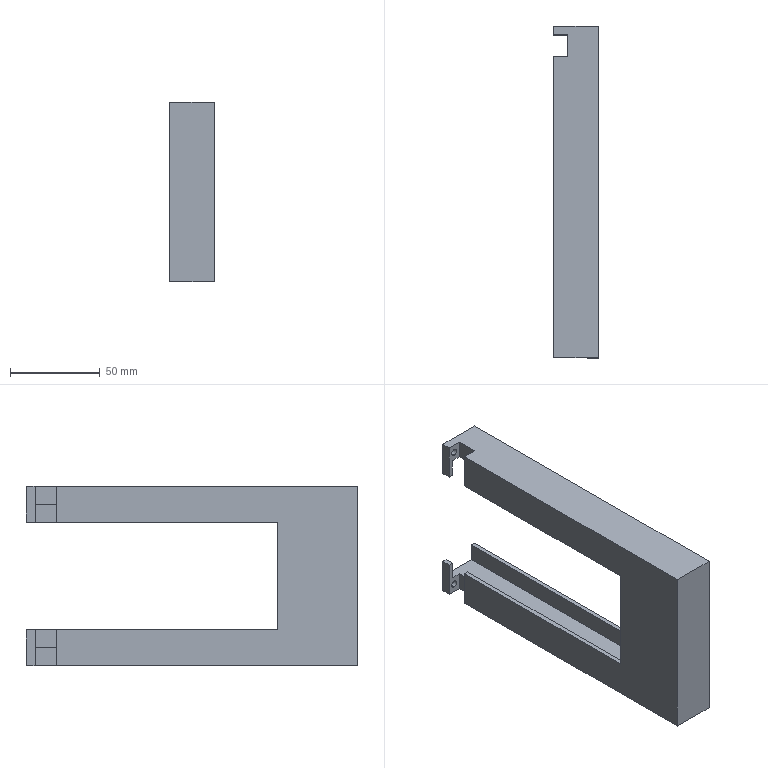Component | SolidWorks | LocatingDie-1_LocatingDieHolder-1 | 1 solid | 34 faces | box 25 x 185 x 100 mm | volume 193854 mm3 | plane 30 | cylinder 4 | commonest cylinder face diameters 4 x4
build123d program:
from build123d import *

# Parameters (mm, degrees)
EXTRUDE1_DEPTH = 25
SKETCH2_W      = 80
SKETCH2_H      = 20
EXTRUDE2_DEPTH = 140
EXTRUDE3_REACH = 140.496
SKETCH3_W      = 8
SKETCH3_H      = 12
EXTRUDE4_REACH = 195.261
SKETCH4_R      = 2


with BuildPart() as part:
    # Sketch1 → Extrude1 (new body)
    with BuildSketch(Plane.XY):
        Polygon((-30, 92.5), (-30, -47.5), (30, -47.5), (30, 92.5), (50, 92.5), (50, -92.5), (-50, -92.5), (-50, 92.5), align=None)
    extrude(amount=EXTRUDE1_DEPTH)

    # Sketch2 → Extrude2 (cut)
    with BuildSketch(Plane(origin=(0, 92.5, 0), x_dir=(1, 0, 0), z_dir=(0, 1, 0))):
        with Locations((0, -12.5)):
            Rectangle(SKETCH2_W, SKETCH2_H)
    extrude(amount=-EXTRUDE2_DEPTH, mode=Mode.SUBTRACT)

    # Extrude3: up to this face of the body (flat: up to its plane)
    extrude3_end = Plane(part.part.faces().sort_by_distance((-50, 0, 12.5))[0])
    # Sketch3 → Extrude3 (cut, up to the picked face)
    with BuildSketch(Plane(origin=(50, 0, 0), x_dir=(0, 0, -1), z_dir=(1, 0, 0)), mode=Mode.PRIVATE) as extrude3_sk1:
        with Locations((-21, 81.5)):
            Rectangle(SKETCH3_W, SKETCH3_H)
    extrude3_tool1 = split(extrude(extrude3_sk1.sketch, amount=-EXTRUDE3_REACH, mode=Mode.PRIVATE), bisect_by=extrude3_end, keep=Keep.BOTH, mode=Mode.PRIVATE)
    add(extrude3_tool1.solids().sort_by(Axis((50, 81.5, 21), (-1, 0, 0)))[0], mode=Mode.SUBTRACT)

    # Sketch4 → Extrude4 (cut, up to next)
    with BuildSketch(Plane(origin=(0, 92.5, 0), x_dir=(1, 0, 0), z_dir=(0, 1, 0)), mode=Mode.PRIVATE) as extrude4_sk1:
        with Locations(Location((45, -21, 0), (0, 0, 180))):
            Circle(SKETCH4_R)
    extrude4_tool1 = extrude(extrude4_sk1.sketch, amount=-EXTRUDE4_REACH, mode=Mode.PRIVATE) & part.part
    # Sketch4 → Extrude4 (cut, up to next)
    with BuildSketch(Plane(origin=(0, 92.5, 0), x_dir=(1, 0, 0), z_dir=(0, 1, 0)), mode=Mode.PRIVATE) as extrude4_sk2:
        with Locations(Location((-45, -21, 0), (0, 0, 180))):
            Circle(SKETCH4_R)
    extrude4_tool2 = extrude(extrude4_sk2.sketch, amount=-EXTRUDE4_REACH, mode=Mode.PRIVATE) & part.part
    add(extrude4_tool1.solids().sort_by_distance((45, 92.5, 21))[0], mode=Mode.SUBTRACT)
    add(extrude4_tool2.solids().sort_by_distance((-45, 92.5, 21))[0], mode=Mode.SUBTRACT)


solid = part.part

# Placed as in the assembly
solid = solid.moved(Location((-19.284, 538.483, 14), (0, -90, 0)))
STEP:
#1=COLOUR_RGB('',0.7922,0.8196,0.9333);
#2=FILL_AREA_STYLE_COLOUR('',#1);
#3=FILL_AREA_STYLE('',(#2));
#4=SURFACE_STYLE_FILL_AREA(#3);
#5=SURFACE_SIDE_STYLE('',(#4));
#6=SURFACE_STYLE_USAGE(.BOTH.,#5);
#7=PRESENTATION_STYLE_ASSIGNMENT((#6));
#8=CARTESIAN_POINT('',(-1.586,24.645,-1.299));
#9=VERTEX_POINT('',#8);
#10=CARTESIAN_POINT('',(-1.586,24.645,-1.142));
#11=VERTEX_POINT('',#10);
#12=CARTESIAN_POINT('',(-1.586,24.645,-1.22));
#13=DIRECTION('',(0.,-1.,0.));
#14=DIRECTION('',(-1.,0.,0.));
#15=AXIS2_PLACEMENT_3D('',#12,#13,#14);
#16=CIRCLE('',#15,0.07874);
#17=EDGE_CURVE('',#9,#11,#16,.T.);
#18=ORIENTED_EDGE('',*,*,#17,.T.);
#19=CARTESIAN_POINT('',(-1.586,24.842,-1.142));
#20=VERTEX_POINT('',#19);
#21=CARTESIAN_POINT('',(-1.586,17.558,-1.142));
#22=DIRECTION('',(-0.,1.,0.));
#23=VECTOR('',#22,39.37);
#24=LINE('',#21,#23);
#25=EDGE_CURVE('',#11,#20,#24,.T.);
#26=ORIENTED_EDGE('',*,*,#25,.T.);
#27=CARTESIAN_POINT('',(-1.586,24.842,-1.299));
#28=VERTEX_POINT('',#27);
#29=CARTESIAN_POINT('',(-1.586,24.842,-1.22));
#30=DIRECTION('',(-0.,1.,0.));
#31=DIRECTION('',(-0.,0.,-1.));
#32=AXIS2_PLACEMENT_3D('',#29,#30,#31);
#33=CIRCLE('',#32,0.07874);
#34=EDGE_CURVE('',#20,#28,#33,.T.);
#35=ORIENTED_EDGE('',*,*,#34,.T.);
#36=CARTESIAN_POINT('',(-1.586,17.558,-1.299));
#37=DIRECTION('',(-0.,1.,0.));
#38=VECTOR('',#37,39.37);
#39=LINE('',#36,#38);
#40=EDGE_CURVE('',#9,#28,#39,.T.);
#41=ORIENTED_EDGE('',*,*,#40,.F.);
#42=EDGE_LOOP('',(#18,#26,#35,#41));
#43=FACE_OUTER_BOUND('',#42,.T.);
#44=CARTESIAN_POINT('',(-1.586,17.558,-1.22));
#45=DIRECTION('',(-0.,1.,0.));
#46=DIRECTION('',(-0.,0.,-1.));
#47=AXIS2_PLACEMENT_3D('',#44,#45,#46);
#48=CYLINDRICAL_SURFACE('',#47,0.07874);
#49=ADVANCED_FACE('',(#43),#48,.F.);
#50=CARTESIAN_POINT('',(-1.586,24.645,2.244));
#51=VERTEX_POINT('',#50);
#52=CARTESIAN_POINT('',(-1.586,24.645,2.402));
#53=VERTEX_POINT('',#52);
#54=CARTESIAN_POINT('',(-1.586,24.645,2.323));
#55=DIRECTION('',(0.,-1.,0.));
#56=DIRECTION('',(-1.,0.,0.));
#57=AXIS2_PLACEMENT_3D('',#54,#55,#56);
#58=CIRCLE('',#57,0.07874);
#59=EDGE_CURVE('',#51,#53,#58,.T.);
#60=ORIENTED_EDGE('',*,*,#59,.T.);
#61=CARTESIAN_POINT('',(-1.586,24.842,2.402));
#62=VERTEX_POINT('',#61);
#63=CARTESIAN_POINT('',(-1.586,17.558,2.402));
#64=DIRECTION('',(-0.,1.,0.));
#65=VECTOR('',#64,39.37);
#66=LINE('',#63,#65);
#67=EDGE_CURVE('',#53,#62,#66,.T.);
#68=ORIENTED_EDGE('',*,*,#67,.T.);
#69=CARTESIAN_POINT('',(-1.586,24.842,2.244));
#70=VERTEX_POINT('',#69);
#71=CARTESIAN_POINT('',(-1.586,24.842,2.323));
#72=DIRECTION('',(-0.,1.,0.));
#73=DIRECTION('',(-0.,0.,-1.));
#74=AXIS2_PLACEMENT_3D('',#71,#72,#73);
#75=CIRCLE('',#74,0.07874);
#76=EDGE_CURVE('',#62,#70,#75,.T.);
#77=ORIENTED_EDGE('',*,*,#76,.T.);
#78=CARTESIAN_POINT('',(-1.586,17.558,2.244));
#79=DIRECTION('',(-0.,1.,0.));
#80=VECTOR('',#79,39.37);
#81=LINE('',#78,#80);
#82=EDGE_CURVE('',#51,#70,#81,.T.);
#83=ORIENTED_EDGE('',*,*,#82,.F.);
#84=EDGE_LOOP('',(#60,#68,#77,#83));
#85=FACE_OUTER_BOUND('',#84,.T.);
#86=CARTESIAN_POINT('',(-1.586,17.558,2.323));
#87=DIRECTION('',(-0.,1.,0.));
#88=DIRECTION('',(-0.,0.,-1.));
#89=AXIS2_PLACEMENT_3D('',#86,#87,#88);
#90=CYLINDRICAL_SURFACE('',#89,0.07874);
#91=ADVANCED_FACE('',(#85),#90,.F.);
#92=CARTESIAN_POINT('',(-1.645,24.842,1.732));
#93=VERTEX_POINT('',#92);
#94=CARTESIAN_POINT('',(-1.645,24.645,1.732));
#95=VERTEX_POINT('',#94);
#96=CARTESIAN_POINT('',(-1.645,19.33,1.732));
#97=DIRECTION('',(0.,-1.,0.));
#98=VECTOR('',#97,39.37);
#99=LINE('',#96,#98);
#100=EDGE_CURVE('',#93,#95,#99,.T.);
#101=ORIENTED_EDGE('',*,*,#100,.T.);
#102=CARTESIAN_POINT('',(-1.743,24.645,1.732));
#103=VERTEX_POINT('',#102);
#104=CARTESIAN_POINT('',(-1.743,24.645,1.732));
#105=DIRECTION('',(-1.,-0.,0.));
#106=VECTOR('',#105,39.37);
#107=LINE('',#104,#106);
#108=EDGE_CURVE('',#95,#103,#107,.T.);
#109=ORIENTED_EDGE('',*,*,#108,.T.);
#110=CARTESIAN_POINT('',(-1.743,24.842,1.732));
#111=VERTEX_POINT('',#110);
#112=CARTESIAN_POINT('',(-1.743,19.33,1.732));
#113=DIRECTION('',(0.,-1.,0.));
#114=VECTOR('',#113,39.37);
#115=LINE('',#112,#114);
#116=EDGE_CURVE('',#111,#103,#115,.T.);
#117=ORIENTED_EDGE('',*,*,#116,.F.);
#118=CARTESIAN_POINT('',(-1.743,24.842,1.732));
#119=DIRECTION('',(1.,0.,-0.));
#120=VECTOR('',#119,39.37);
#121=LINE('',#118,#120);
#122=EDGE_CURVE('',#111,#93,#121,.T.);
#123=ORIENTED_EDGE('',*,*,#122,.T.);
#124=EDGE_LOOP('',(#101,#109,#117,#123));
#125=FACE_OUTER_BOUND('',#124,.T.);
#126=CARTESIAN_POINT('',(-1.743,19.33,1.732));
#127=DIRECTION('',(0.,0.,1.));
#128=DIRECTION('',(-0.,1.,-0.));
#129=AXIS2_PLACEMENT_3D('',#126,#127,#128);
#130=PLANE('',#129);
#131=ADVANCED_FACE('',(#125),#130,.F.);
#132=CARTESIAN_POINT('',(-1.743,24.645,-0.6299));
#133=VERTEX_POINT('',#132);
#134=CARTESIAN_POINT('',(-1.743,24.842,-0.6299));
#135=VERTEX_POINT('',#134);
#136=CARTESIAN_POINT('',(-1.743,24.842,-0.6299));
#137=DIRECTION('',(-0.,1.,-0.));
#138=VECTOR('',#137,39.37);
#139=LINE('',#136,#138);
#140=EDGE_CURVE('',#133,#135,#139,.T.);
#141=ORIENTED_EDGE('',*,*,#140,.F.);
#142=CARTESIAN_POINT('',(-1.645,24.645,-0.6299));
#143=VERTEX_POINT('',#142);
#144=CARTESIAN_POINT('',(-1.743,24.645,-0.6299));
#145=DIRECTION('',(1.,0.,-0.));
#146=VECTOR('',#145,39.37);
#147=LINE('',#144,#146);
#148=EDGE_CURVE('',#133,#143,#147,.T.);
#149=ORIENTED_EDGE('',*,*,#148,.T.);
#150=CARTESIAN_POINT('',(-1.645,24.842,-0.6299));
#151=VERTEX_POINT('',#150);
#152=CARTESIAN_POINT('',(-1.645,24.842,-0.6299));
#153=DIRECTION('',(-0.,1.,-0.));
#154=VECTOR('',#153,39.37);
#155=LINE('',#152,#154);
#156=EDGE_CURVE('',#143,#151,#155,.T.);
#157=ORIENTED_EDGE('',*,*,#156,.T.);
#158=CARTESIAN_POINT('',(-1.743,24.842,-0.6299));
#159=DIRECTION('',(1.,0.,-0.));
#160=VECTOR('',#159,39.37);
#161=LINE('',#158,#160);
#162=EDGE_CURVE('',#135,#151,#161,.T.);
#163=ORIENTED_EDGE('',*,*,#162,.F.);
#164=EDGE_LOOP('',(#141,#149,#157,#163));
#165=FACE_OUTER_BOUND('',#164,.T.);
#166=CARTESIAN_POINT('',(-1.743,24.842,-0.6299));
#167=DIRECTION('',(-0.,-0.,-1.));
#168=DIRECTION('',(0.,-1.,0.));
#169=AXIS2_PLACEMENT_3D('',#166,#167,#168);
#170=PLANE('',#169);
#171=ADVANCED_FACE('',(#165),#170,.F.);
#172=CARTESIAN_POINT('',(-1.743,24.645,-1.417));
#173=VERTEX_POINT('',#172);
#174=CARTESIAN_POINT('',(-1.743,24.645,-1.985));
#175=DIRECTION('',(0.,0.,1.));
#176=VECTOR('',#175,39.37);
#177=LINE('',#174,#176);
#178=EDGE_CURVE('',#173,#133,#177,.T.);
#179=ORIENTED_EDGE('',*,*,#178,.T.);
#180=ORIENTED_EDGE('',*,*,#140,.T.);
#181=CARTESIAN_POINT('',(-1.743,24.842,-1.417));
#182=VERTEX_POINT('',#181);
#183=CARTESIAN_POINT('',(-1.743,24.842,-1.417));
#184=DIRECTION('',(-0.,-0.,-1.));
#185=VECTOR('',#184,39.37);
#186=LINE('',#183,#185);
#187=EDGE_CURVE('',#135,#182,#186,.T.);
#188=ORIENTED_EDGE('',*,*,#187,.T.);
#189=CARTESIAN_POINT('',(-1.743,24.842,-1.417));
#190=DIRECTION('',(0.,-1.,0.));
#191=VECTOR('',#190,39.37);
#192=LINE('',#189,#191);
#193=EDGE_CURVE('',#182,#173,#192,.T.);
#194=ORIENTED_EDGE('',*,*,#193,.T.);
#195=EDGE_LOOP('',(#179,#180,#188,#194));
#196=FACE_OUTER_BOUND('',#195,.T.);
#197=CARTESIAN_POINT('',(-1.743,17.558,-1.417));
#198=DIRECTION('',(-1.,-0.,0.));
#199=DIRECTION('',(0.,0.,1.));
#200=AXIS2_PLACEMENT_3D('',#197,#198,#199);
#201=PLANE('',#200);
#202=ADVANCED_FACE('',(#196),#201,.T.);
#203=CARTESIAN_POINT('',(-1.743,24.645,2.52));
#204=VERTEX_POINT('',#203);
#205=CARTESIAN_POINT('',(-1.743,24.645,-1.985));
#206=DIRECTION('',(0.,0.,1.));
#207=VECTOR('',#206,39.37);
#208=LINE('',#205,#207);
#209=EDGE_CURVE('',#103,#204,#208,.T.);
#210=ORIENTED_EDGE('',*,*,#209,.T.);
#211=CARTESIAN_POINT('',(-1.743,24.842,2.52));
#212=VERTEX_POINT('',#211);
#213=CARTESIAN_POINT('',(-1.743,24.842,2.52));
#214=DIRECTION('',(-0.,1.,-0.));
#215=VECTOR('',#214,39.37);
#216=LINE('',#213,#215);
#217=EDGE_CURVE('',#204,#212,#216,.T.);
#218=ORIENTED_EDGE('',*,*,#217,.T.);
#219=CARTESIAN_POINT('',(-1.743,24.842,1.732));
#220=DIRECTION('',(-0.,0.,-1.));
#221=VECTOR('',#220,39.37);
#222=LINE('',#219,#221);
#223=EDGE_CURVE('',#212,#111,#222,.T.);
#224=ORIENTED_EDGE('',*,*,#223,.T.);
#225=ORIENTED_EDGE('',*,*,#116,.T.);
#226=EDGE_LOOP('',(#210,#218,#224,#225));
#227=FACE_OUTER_BOUND('',#226,.T.);
#228=CARTESIAN_POINT('',(-1.743,17.558,-1.417));
#229=DIRECTION('',(-1.,-0.,0.));
#230=DIRECTION('',(0.,0.,1.));
#231=AXIS2_PLACEMENT_3D('',#228,#229,#230);
#232=PLANE('',#231);
#233=ADVANCED_FACE('',(#227),#232,.T.);
#234=ORIENTED_EDGE('',*,*,#156,.F.);
#235=CARTESIAN_POINT('',(-1.645,24.645,-1.024));
#236=VERTEX_POINT('',#235);
#237=CARTESIAN_POINT('',(-1.645,24.645,-1.024));
#238=DIRECTION('',(-0.,-0.,-1.));
#239=VECTOR('',#238,39.37);
#240=LINE('',#237,#239);
#241=EDGE_CURVE('',#143,#236,#240,.T.);
#242=ORIENTED_EDGE('',*,*,#241,.T.);
#243=CARTESIAN_POINT('',(-1.645,24.842,-1.024));
#244=VERTEX_POINT('',#243);
#245=CARTESIAN_POINT('',(-1.645,16.084,-1.024));
#246=DIRECTION('',(-0.,1.,-0.));
#247=VECTOR('',#246,39.37);
#248=LINE('',#245,#247);
#249=EDGE_CURVE('',#236,#244,#248,.T.);
#250=ORIENTED_EDGE('',*,*,#249,.T.);
#251=CARTESIAN_POINT('',(-1.645,24.842,-1.024));
#252=DIRECTION('',(0.,0.,1.));
#253=VECTOR('',#252,39.37);
#254=LINE('',#251,#253);
#255=EDGE_CURVE('',#244,#151,#254,.T.);
#256=ORIENTED_EDGE('',*,*,#255,.T.);
#257=EDGE_LOOP('',(#234,#242,#250,#256));
#258=FACE_OUTER_BOUND('',#257,.T.);
#259=CARTESIAN_POINT('',(-1.645,16.084,-1.024));
#260=DIRECTION('',(-1.,-0.,0.));
#261=DIRECTION('',(0.,0.,1.));
#262=AXIS2_PLACEMENT_3D('',#259,#260,#261);
#263=PLANE('',#262);
#264=ADVANCED_FACE('',(#258),#263,.F.);
#265=CARTESIAN_POINT('',(-1.645,24.645,2.126));
#266=VERTEX_POINT('',#265);
#267=CARTESIAN_POINT('',(-1.645,24.842,2.126));
#268=VERTEX_POINT('',#267);
#269=CARTESIAN_POINT('',(-1.645,16.084,2.126));
#270=DIRECTION('',(-0.,1.,-0.));
#271=VECTOR('',#270,39.37);
#272=LINE('',#269,#271);
#273=EDGE_CURVE('',#266,#268,#272,.T.);
#274=ORIENTED_EDGE('',*,*,#273,.F.);
#275=CARTESIAN_POINT('',(-1.645,24.645,-1.024));
#276=DIRECTION('',(-0.,-0.,-1.));
#277=VECTOR('',#276,39.37);
#278=LINE('',#275,#277);
#279=EDGE_CURVE('',#266,#95,#278,.T.);
#280=ORIENTED_EDGE('',*,*,#279,.T.);
#281=ORIENTED_EDGE('',*,*,#100,.F.);
#282=CARTESIAN_POINT('',(-1.645,24.842,-1.024));
#283=DIRECTION('',(0.,0.,1.));
#284=VECTOR('',#283,39.37);
#285=LINE('',#282,#284);
#286=EDGE_CURVE('',#93,#268,#285,.T.);
#287=ORIENTED_EDGE('',*,*,#286,.T.);
#288=EDGE_LOOP('',(#274,#280,#281,#287));
#289=FACE_OUTER_BOUND('',#288,.T.);
#290=CARTESIAN_POINT('',(-1.645,16.084,-1.024));
#291=DIRECTION('',(-1.,-0.,0.));
#292=DIRECTION('',(0.,0.,1.));
#293=AXIS2_PLACEMENT_3D('',#290,#291,#292);
#294=PLANE('',#293);
#295=ADVANCED_FACE('',(#289),#294,.F.);
#296=CARTESIAN_POINT('',(-1.743,24.173,1.732));
#297=VERTEX_POINT('',#296);
#298=CARTESIAN_POINT('',(-1.743,19.33,1.732));
#299=VERTEX_POINT('',#298);
#300=CARTESIAN_POINT('',(-1.743,19.33,1.732));
#301=DIRECTION('',(0.,-1.,0.));
#302=VECTOR('',#301,39.37);
#303=LINE('',#300,#302);
#304=EDGE_CURVE('',#297,#299,#303,.T.);
#305=ORIENTED_EDGE('',*,*,#304,.F.);
#306=CARTESIAN_POINT('',(-1.645,24.173,1.732));
#307=VERTEX_POINT('',#306);
#308=CARTESIAN_POINT('',(-1.743,24.173,1.732));
#309=DIRECTION('',(1.,0.,-0.));
#310=VECTOR('',#309,39.37);
#311=LINE('',#308,#310);
#312=EDGE_CURVE('',#297,#307,#311,.T.);
#313=ORIENTED_EDGE('',*,*,#312,.T.);
#314=CARTESIAN_POINT('',(-1.645,19.33,1.732));
#315=VERTEX_POINT('',#314);
#316=CARTESIAN_POINT('',(-1.645,19.33,1.732));
#317=DIRECTION('',(0.,-1.,0.));
#318=VECTOR('',#317,39.37);
#319=LINE('',#316,#318);
#320=EDGE_CURVE('',#307,#315,#319,.T.);
#321=ORIENTED_EDGE('',*,*,#320,.T.);
#322=CARTESIAN_POINT('',(-1.743,19.33,1.732));
#323=DIRECTION('',(1.,0.,-0.));
#324=VECTOR('',#323,39.37);
#325=LINE('',#322,#324);
#326=EDGE_CURVE('',#299,#315,#325,.T.);
#327=ORIENTED_EDGE('',*,*,#326,.F.);
#328=EDGE_LOOP('',(#305,#313,#321,#327));
#329=FACE_OUTER_BOUND('',#328,.T.);
#330=CARTESIAN_POINT('',(-1.743,19.33,1.732));
#331=DIRECTION('',(0.,0.,1.));
#332=DIRECTION('',(-0.,1.,-0.));
#333=AXIS2_PLACEMENT_3D('',#330,#331,#332);
#334=PLANE('',#333);
#335=ADVANCED_FACE('',(#329),#334,.F.);
#336=CARTESIAN_POINT('',(-1.645,19.33,-0.6299));
#337=VERTEX_POINT('',#336);
#338=CARTESIAN_POINT('',(-1.645,24.173,-0.6299));
#339=VERTEX_POINT('',#338);
#340=CARTESIAN_POINT('',(-1.645,24.842,-0.6299));
#341=DIRECTION('',(-0.,1.,-0.));
#342=VECTOR('',#341,39.37);
#343=LINE('',#340,#342);
#344=EDGE_CURVE('',#337,#339,#343,.T.);
#345=ORIENTED_EDGE('',*,*,#344,.T.);
#346=CARTESIAN_POINT('',(-1.743,24.173,-0.6299));
#347=VERTEX_POINT('',#346);
#348=CARTESIAN_POINT('',(-1.743,24.173,-0.6299));
#349=DIRECTION('',(-1.,-0.,0.));
#350=VECTOR('',#349,39.37);
#351=LINE('',#348,#350);
#352=EDGE_CURVE('',#339,#347,#351,.T.);
#353=ORIENTED_EDGE('',*,*,#352,.T.);
#354=CARTESIAN_POINT('',(-1.743,19.33,-0.6299));
#355=VERTEX_POINT('',#354);
#356=CARTESIAN_POINT('',(-1.743,24.842,-0.6299));
#357=DIRECTION('',(-0.,1.,-0.));
#358=VECTOR('',#357,39.37);
#359=LINE('',#356,#358);
#360=EDGE_CURVE('',#355,#347,#359,.T.);
#361=ORIENTED_EDGE('',*,*,#360,.F.);
#362=CARTESIAN_POINT('',(-1.743,19.33,-0.6299));
#363=DIRECTION('',(1.,0.,-0.));
#364=VECTOR('',#363,39.37);
#365=LINE('',#362,#364);
#366=EDGE_CURVE('',#355,#337,#365,.T.);
#367=ORIENTED_EDGE('',*,*,#366,.T.);
#368=EDGE_LOOP('',(#345,#353,#361,#367));
#369=FACE_OUTER_BOUND('',#368,.T.);
#370=CARTESIAN_POINT('',(-1.743,24.842,-0.6299));
#371=DIRECTION('',(-0.,-0.,-1.));
#372=DIRECTION('',(0.,-1.,0.));
#373=AXIS2_PLACEMENT_3D('',#370,#371,#372);
#374=PLANE('',#373);
#375=ADVANCED_FACE('',(#369),#374,.F.);
#376=CARTESIAN_POINT('',(-1.428,24.645,-1.417));
#377=VERTEX_POINT('',#376);
#378=CARTESIAN_POINT('',(-1.428,24.173,-1.417));
#379=VERTEX_POINT('',#378);
#380=CARTESIAN_POINT('',(-1.428,24.645,-1.417));
#381=DIRECTION('',(0.,-1.,0.));
#382=VECTOR('',#381,39.37);
#383=LINE('',#380,#382);
#384=EDGE_CURVE('',#377,#379,#383,.T.);
#385=ORIENTED_EDGE('',*,*,#384,.F.);
#386=CARTESIAN_POINT('',(-1.743,24.645,-1.417));
#387=DIRECTION('',(1.,0.,-0.));
#388=VECTOR('',#387,39.37);
#389=LINE('',#386,#388);
#390=EDGE_CURVE('',#173,#377,#389,.T.);
#391=ORIENTED_EDGE('',*,*,#390,.F.);
#392=ORIENTED_EDGE('',*,*,#193,.F.);
#393=CARTESIAN_POINT('',(-0.7592,24.842,-1.417));
#394=VERTEX_POINT('',#393);
#395=CARTESIAN_POINT('',(-1.743,24.842,-1.417));
#396=DIRECTION('',(1.,0.,-0.));
#397=VECTOR('',#396,39.37);
#398=LINE('',#395,#397);
#399=EDGE_CURVE('',#182,#394,#398,.T.);
#400=ORIENTED_EDGE('',*,*,#399,.T.);
#401=CARTESIAN_POINT('',(-0.7592,17.558,-1.417));
#402=VERTEX_POINT('',#401);
#403=CARTESIAN_POINT('',(-0.7592,24.842,-1.417));
#404=DIRECTION('',(0.,-1.,0.));
#405=VECTOR('',#404,39.37);
#406=LINE('',#403,#405);
#407=EDGE_CURVE('',#394,#402,#406,.T.);
#408=ORIENTED_EDGE('',*,*,#407,.T.);
#409=CARTESIAN_POINT('',(-1.743,17.558,-1.417));
#410=VERTEX_POINT('',#409);
#411=CARTESIAN_POINT('',(-1.743,17.558,-1.417));
#412=DIRECTION('',(1.,0.,-0.));
#413=VECTOR('',#412,39.37);
#414=LINE('',#411,#413);
#415=EDGE_CURVE('',#410,#402,#414,.T.);
#416=ORIENTED_EDGE('',*,*,#415,.F.);
#417=CARTESIAN_POINT('',(-1.743,24.173,-1.417));
#418=VERTEX_POINT('',#417);
#419=CARTESIAN_POINT('',(-1.743,24.842,-1.417));
#420=DIRECTION('',(0.,-1.,0.));
#421=VECTOR('',#420,39.37);
#422=LINE('',#419,#421);
#423=EDGE_CURVE('',#418,#410,#422,.T.);
#424=ORIENTED_EDGE('',*,*,#423,.F.);
#425=CARTESIAN_POINT('',(-1.743,24.173,-1.417));
#426=DIRECTION('',(-1.,-0.,0.));
#427=VECTOR('',#426,39.37);
#428=LINE('',#425,#427);
#429=EDGE_CURVE('',#379,#418,#428,.T.);
#430=ORIENTED_EDGE('',*,*,#429,.F.);
#431=EDGE_LOOP('',(#385,#391,#392,#400,#408,#416,#424,#430));
#432=FACE_OUTER_BOUND('',#431,.T.);
#433=CARTESIAN_POINT('',(-1.743,24.842,-1.417));
#434=DIRECTION('',(0.,0.,1.));
#435=DIRECTION('',(1.,0.,-0.));
#436=AXIS2_PLACEMENT_3D('',#433,#434,#435);
#437=PLANE('',#436);
#438=ADVANCED_FACE('',(#432),#437,.F.);
#439=CARTESIAN_POINT('',(-0.7592,17.558,2.52));
#440=VERTEX_POINT('',#439);
#441=CARTESIAN_POINT('',(-0.7592,17.558,-1.417));
#442=DIRECTION('',(0.,0.,1.));
#443=VECTOR('',#442,39.37);
#444=LINE('',#441,#443);
#445=EDGE_CURVE('',#402,#440,#444,.T.);
#446=ORIENTED_EDGE('',*,*,#445,.T.);
#447=CARTESIAN_POINT('',(-1.743,17.558,2.52));
#448=VERTEX_POINT('',#447);
#449=CARTESIAN_POINT('',(-1.743,17.558,2.52));
#450=DIRECTION('',(1.,0.,-0.));
#451=VECTOR('',#450,39.37);
#452=LINE('',#449,#451);
#453=EDGE_CURVE('',#448,#440,#452,.T.);
#454=ORIENTED_EDGE('',*,*,#453,.F.);
#455=CARTESIAN_POINT('',(-1.743,17.558,-1.417));
#456=DIRECTION('',(0.,0.,1.));
#457=VECTOR('',#456,39.37);
#458=LINE('',#455,#457);
#459=EDGE_CURVE('',#410,#448,#458,.T.);
#460=ORIENTED_EDGE('',*,*,#459,.F.);
#461=ORIENTED_EDGE('',*,*,#415,.T.);
#462=EDGE_LOOP('',(#446,#454,#460,#461));
#463=FACE_OUTER_BOUND('',#462,.T.);
#464=CARTESIAN_POINT('',(-1.743,17.558,-1.417));
#465=DIRECTION('',(-0.,1.,-0.));
#466=DIRECTION('',(-1.,-0.,0.));
#467=AXIS2_PLACEMENT_3D('',#464,#465,#466);
#468=PLANE('',#467);
#469=ADVANCED_FACE('',(#463),#468,.F.);
#470=ORIENTED_EDGE('',*,*,#217,.F.);
#471=CARTESIAN_POINT('',(-1.428,24.645,2.52));
#472=VERTEX_POINT('',#471);
#473=CARTESIAN_POINT('',(-1.743,24.645,2.52));
#474=DIRECTION('',(-1.,-0.,0.));
#475=VECTOR('',#474,39.37);
#476=LINE('',#473,#475);
#477=EDGE_CURVE('',#472,#204,#476,.T.);
#478=ORIENTED_EDGE('',*,*,#477,.F.);
#479=CARTESIAN_POINT('',(-1.428,24.173,2.52));
#480=VERTEX_POINT('',#479);
#481=CARTESIAN_POINT('',(-1.428,24.645,2.52));
#482=DIRECTION('',(-0.,1.,-0.));
#483=VECTOR('',#482,39.37);
#484=LINE('',#481,#483);
#485=EDGE_CURVE('',#480,#472,#484,.T.);
#486=ORIENTED_EDGE('',*,*,#485,.F.);
#487=CARTESIAN_POINT('',(-1.743,24.173,2.52));
#488=VERTEX_POINT('',#487);
#489=CARTESIAN_POINT('',(-1.743,24.173,2.52));
#490=DIRECTION('',(1.,0.,-0.));
#491=VECTOR('',#490,39.37);
#492=LINE('',#489,#491);
#493=EDGE_CURVE('',#488,#480,#492,.T.);
#494=ORIENTED_EDGE('',*,*,#493,.F.);
#495=CARTESIAN_POINT('',(-1.743,24.842,2.52));
#496=DIRECTION('',(-0.,1.,-0.));
#497=VECTOR('',#496,39.37);
#498=LINE('',#495,#497);
#499=EDGE_CURVE('',#448,#488,#498,.T.);
#500=ORIENTED_EDGE('',*,*,#499,.F.);
#501=ORIENTED_EDGE('',*,*,#453,.T.);
#502=CARTESIAN_POINT('',(-0.7592,24.842,2.52));
#503=VERTEX_POINT('',#502);
#504=CARTESIAN_POINT('',(-0.7592,24.842,2.52));
#505=DIRECTION('',(-0.,1.,-0.));
#506=VECTOR('',#505,39.37);
#507=LINE('',#504,#506);
#508=EDGE_CURVE('',#440,#503,#507,.T.);
#509=ORIENTED_EDGE('',*,*,#508,.T.);
#510=CARTESIAN_POINT('',(-1.743,24.842,2.52));
#511=DIRECTION('',(1.,0.,-0.));
#512=VECTOR('',#511,39.37);
#513=LINE('',#510,#512);
#514=EDGE_CURVE('',#212,#503,#513,.T.);
#515=ORIENTED_EDGE('',*,*,#514,.F.);
#516=EDGE_LOOP('',(#470,#478,#486,#494,#500,#501,#509,#515));
#517=FACE_OUTER_BOUND('',#516,.T.);
#518=CARTESIAN_POINT('',(-1.743,24.842,2.52));
#519=DIRECTION('',(-0.,-0.,-1.));
#520=DIRECTION('',(-1.,-0.,0.));
#521=AXIS2_PLACEMENT_3D('',#518,#519,#520);
#522=PLANE('',#521);
#523=ADVANCED_FACE('',(#517),#522,.F.);
#524=CARTESIAN_POINT('',(-1.586,24.842,2.323));
#525=DIRECTION('',(-0.,1.,0.));
#526=DIRECTION('',(-0.,0.,-1.));
#527=AXIS2_PLACEMENT_3D('',#524,#525,#526);
#528=CIRCLE('',#527,0.07874);
#529=EDGE_CURVE('',#70,#62,#528,.T.);
#530=ORIENTED_EDGE('',*,*,#529,.F.);
#531=ORIENTED_EDGE('',*,*,#76,.F.);
#532=EDGE_LOOP('',(#530,#531));
#533=FACE_BOUND('',#532,.T.);
#534=CARTESIAN_POINT('',(-0.8576,24.842,2.126));
#535=VERTEX_POINT('',#534);
#536=CARTESIAN_POINT('',(-0.8576,24.842,2.126));
#537=DIRECTION('',(1.,0.,-0.));
#538=VECTOR('',#537,39.37);
#539=LINE('',#536,#538);
#540=EDGE_CURVE('',#268,#535,#539,.T.);
#541=ORIENTED_EDGE('',*,*,#540,.F.);
#542=ORIENTED_EDGE('',*,*,#286,.F.);
#543=ORIENTED_EDGE('',*,*,#122,.F.);
#544=ORIENTED_EDGE('',*,*,#223,.F.);
#545=ORIENTED_EDGE('',*,*,#514,.T.);
#546=CARTESIAN_POINT('',(-0.7592,24.842,1.732));
#547=VERTEX_POINT('',#546);
#548=CARTESIAN_POINT('',(-0.7592,24.842,1.732));
#549=DIRECTION('',(-0.,0.,-1.));
#550=VECTOR('',#549,39.37);
#551=LINE('',#548,#550);
#552=EDGE_CURVE('',#503,#547,#551,.T.);
#553=ORIENTED_EDGE('',*,*,#552,.T.);
#554=CARTESIAN_POINT('',(-0.8576,24.842,1.732));
#555=VERTEX_POINT('',#554);
#556=CARTESIAN_POINT('',(-1.743,24.842,1.732));
#557=DIRECTION('',(1.,0.,-0.));
#558=VECTOR('',#557,39.37);
#559=LINE('',#556,#558);
#560=EDGE_CURVE('',#555,#547,#559,.T.);
#561=ORIENTED_EDGE('',*,*,#560,.F.);
#562=CARTESIAN_POINT('',(-0.8576,24.842,-1.024));
#563=DIRECTION('',(-0.,-0.,-1.));
#564=VECTOR('',#563,39.37);
#565=LINE('',#562,#564);
#566=EDGE_CURVE('',#535,#555,#565,.T.);
#567=ORIENTED_EDGE('',*,*,#566,.F.);
#568=EDGE_LOOP('',(#541,#542,#543,#544,#545,#553,#561,#567));
#569=FACE_OUTER_BOUND('',#568,.T.);
#570=CARTESIAN_POINT('',(-1.743,24.842,1.732));
#571=DIRECTION('',(0.,-1.,-0.));
#572=DIRECTION('',(0.,-0.,1.));
#573=AXIS2_PLACEMENT_3D('',#570,#571,#572);
#574=PLANE('',#573);
#575=ADVANCED_FACE('',(#533,#569),#574,.F.);
#576=CARTESIAN_POINT('',(-0.8576,19.33,1.732));
#577=VERTEX_POINT('',#576);
#578=CARTESIAN_POINT('',(-0.7592,19.33,1.732));
#579=VERTEX_POINT('',#578);
#580=CARTESIAN_POINT('',(-1.743,19.33,1.732));
#581=DIRECTION('',(1.,0.,-0.));
#582=VECTOR('',#581,39.37);
#583=LINE('',#580,#582);
#584=EDGE_CURVE('',#577,#579,#583,.T.);
#585=ORIENTED_EDGE('',*,*,#584,.F.);
#586=CARTESIAN_POINT('',(-0.8576,19.33,1.732));
#587=DIRECTION('',(-0.,1.,-0.));
#588=VECTOR('',#587,39.37);
#589=LINE('',#586,#588);
#590=EDGE_CURVE('',#577,#555,#589,.T.);
#591=ORIENTED_EDGE('',*,*,#590,.T.);
#592=ORIENTED_EDGE('',*,*,#560,.T.);
#593=CARTESIAN_POINT('',(-0.7592,19.33,1.732));
#594=DIRECTION('',(0.,-1.,0.));
#595=VECTOR('',#594,39.37);
#596=LINE('',#593,#595);
#597=EDGE_CURVE('',#547,#579,#596,.T.);
#598=ORIENTED_EDGE('',*,*,#597,.T.);
#599=EDGE_LOOP('',(#585,#591,#592,#598));
#600=FACE_OUTER_BOUND('',#599,.T.);
#601=CARTESIAN_POINT('',(-1.743,19.33,1.732));
#602=DIRECTION('',(0.,0.,1.));
#603=DIRECTION('',(-0.,1.,-0.));
#604=AXIS2_PLACEMENT_3D('',#601,#602,#603);
#605=PLANE('',#604);
#606=ADVANCED_FACE('',(#600),#605,.F.);
#607=CARTESIAN_POINT('',(-0.8576,19.33,-0.6299));
#608=VERTEX_POINT('',#607);
#609=CARTESIAN_POINT('',(-0.7592,19.33,-0.6299));
#610=VERTEX_POINT('',#609);
#611=CARTESIAN_POINT('',(-1.743,19.33,-0.6299));
#612=DIRECTION('',(1.,0.,-0.));
#613=VECTOR('',#612,39.37);
#614=LINE('',#611,#613);
#615=EDGE_CURVE('',#608,#610,#614,.T.);
#616=ORIENTED_EDGE('',*,*,#615,.F.);
#617=CARTESIAN_POINT('',(-0.8576,19.33,-1.024));
#618=VERTEX_POINT('',#617);
#619=CARTESIAN_POINT('',(-0.8576,19.33,-1.024));
#620=DIRECTION('',(-0.,-0.,-1.));
#621=VECTOR('',#620,39.37);
#622=LINE('',#619,#621);
#623=EDGE_CURVE('',#608,#618,#622,.T.);
#624=ORIENTED_EDGE('',*,*,#623,.T.);
#625=CARTESIAN_POINT('',(-1.645,19.33,-1.024));
#626=VERTEX_POINT('',#625);
#627=CARTESIAN_POINT('',(-0.8576,19.33,-1.024));
#628=DIRECTION('',(-1.,-0.,0.));
#629=VECTOR('',#628,39.37);
#630=LINE('',#627,#629);
#631=EDGE_CURVE('',#618,#626,#630,.T.);
#632=ORIENTED_EDGE('',*,*,#631,.T.);
#633=CARTESIAN_POINT('',(-1.645,19.33,-1.024));
#634=DIRECTION('',(0.,0.,1.));
#635=VECTOR('',#634,39.37);
#636=LINE('',#633,#635);
#637=EDGE_CURVE('',#626,#337,#636,.T.);
#638=ORIENTED_EDGE('',*,*,#637,.T.);
#639=ORIENTED_EDGE('',*,*,#366,.F.);
#640=CARTESIAN_POINT('',(-1.743,19.33,-0.6299));
#641=DIRECTION('',(-0.,-0.,-1.));
#642=VECTOR('',#641,39.37);
#643=LINE('',#640,#642);
#644=EDGE_CURVE('',#299,#355,#643,.T.);
#645=ORIENTED_EDGE('',*,*,#644,.F.);
#646=ORIENTED_EDGE('',*,*,#326,.T.);
#647=CARTESIAN_POINT('',(-1.645,19.33,2.126));
#648=VERTEX_POINT('',#647);
#649=CARTESIAN_POINT('',(-1.645,19.33,-1.024));
#650=DIRECTION('',(0.,0.,1.));
#651=VECTOR('',#650,39.37);
#652=LINE('',#649,#651);
#653=EDGE_CURVE('',#315,#648,#652,.T.);
#654=ORIENTED_EDGE('',*,*,#653,.T.);
#655=CARTESIAN_POINT('',(-0.8576,19.33,2.126));
#656=VERTEX_POINT('',#655);
#657=CARTESIAN_POINT('',(-0.8576,19.33,2.126));
#658=DIRECTION('',(1.,0.,-0.));
#659=VECTOR('',#658,39.37);
#660=LINE('',#657,#659);
#661=EDGE_CURVE('',#648,#656,#660,.T.);
#662=ORIENTED_EDGE('',*,*,#661,.T.);
#663=CARTESIAN_POINT('',(-0.8576,19.33,-1.024));
#664=DIRECTION('',(-0.,-0.,-1.));
#665=VECTOR('',#664,39.37);
#666=LINE('',#663,#665);
#667=EDGE_CURVE('',#656,#577,#666,.T.);
#668=ORIENTED_EDGE('',*,*,#667,.T.);
#669=ORIENTED_EDGE('',*,*,#584,.T.);
#670=CARTESIAN_POINT('',(-0.7592,19.33,-0.6299));
#671=DIRECTION('',(-0.,-0.,-1.));
#672=VECTOR('',#671,39.37);
#673=LINE('',#670,#672);
#674=EDGE_CURVE('',#579,#610,#673,.T.);
#675=ORIENTED_EDGE('',*,*,#674,.T.);
#676=EDGE_LOOP('',(#616,#624,#632,#638,#639,#645,#646,#654,#662,#668,#669,#675));
#677=FACE_OUTER_BOUND('',#676,.T.);
#678=CARTESIAN_POINT('',(-1.743,19.33,-0.6299));
#679=DIRECTION('',(0.,-1.,0.));
#680=DIRECTION('',(1.,0.,-0.));
#681=AXIS2_PLACEMENT_3D('',#678,#679,#680);
#682=PLANE('',#681);
#683=ADVANCED_FACE('',(#677),#682,.F.);
#684=CARTESIAN_POINT('',(-0.8576,24.842,-0.6299));
#685=VERTEX_POINT('',#684);
#686=CARTESIAN_POINT('',(-0.7592,24.842,-0.6299));
#687=VERTEX_POINT('',#686);
#688=CARTESIAN_POINT('',(-1.743,24.842,-0.6299));
#689=DIRECTION('',(1.,0.,-0.));
#690=VECTOR('',#689,39.37);
#691=LINE('',#688,#690);
#692=EDGE_CURVE('',#685,#687,#691,.T.);
#693=ORIENTED_EDGE('',*,*,#692,.F.);
#694=CARTESIAN_POINT('',(-0.8576,24.842,-0.6299));
#695=DIRECTION('',(0.,-1.,0.));
#696=VECTOR('',#695,39.37);
#697=LINE('',#694,#696);
#698=EDGE_CURVE('',#685,#608,#697,.T.);
#699=ORIENTED_EDGE('',*,*,#698,.T.);
#700=ORIENTED_EDGE('',*,*,#615,.T.);
#701=CARTESIAN_POINT('',(-0.7592,24.842,-0.6299));
#702=DIRECTION('',(-0.,1.,-0.));
#703=VECTOR('',#702,39.37);
#704=LINE('',#701,#703);
#705=EDGE_CURVE('',#610,#687,#704,.T.);
#706=ORIENTED_EDGE('',*,*,#705,.T.);
#707=EDGE_LOOP('',(#693,#699,#700,#706));
#708=FACE_OUTER_BOUND('',#707,.T.);
#709=CARTESIAN_POINT('',(-1.743,24.842,-0.6299));
#710=DIRECTION('',(-0.,-0.,-1.));
#711=DIRECTION('',(0.,-1.,0.));
#712=AXIS2_PLACEMENT_3D('',#709,#710,#711);
#713=PLANE('',#712);
#714=ADVANCED_FACE('',(#708),#713,.F.);
#715=CARTESIAN_POINT('',(-1.586,24.842,-1.22));
#716=DIRECTION('',(-0.,1.,0.));
#717=DIRECTION('',(-0.,0.,-1.));
#718=AXIS2_PLACEMENT_3D('',#715,#716,#717);
#719=CIRCLE('',#718,0.07874);
#720=EDGE_CURVE('',#28,#20,#719,.T.);
#721=ORIENTED_EDGE('',*,*,#720,.F.);
#722=ORIENTED_EDGE('',*,*,#34,.F.);
#723=EDGE_LOOP('',(#721,#722));
#724=FACE_BOUND('',#723,.T.);
#725=ORIENTED_EDGE('',*,*,#162,.T.);
#726=ORIENTED_EDGE('',*,*,#255,.F.);
#727=CARTESIAN_POINT('',(-0.8576,24.842,-1.024));
#728=VERTEX_POINT('',#727);
#729=CARTESIAN_POINT('',(-0.8576,24.842,-1.024));
#730=DIRECTION('',(-1.,-0.,0.));
#731=VECTOR('',#730,39.37);
#732=LINE('',#729,#731);
#733=EDGE_CURVE('',#728,#244,#732,.T.);
#734=ORIENTED_EDGE('',*,*,#733,.F.);
#735=CARTESIAN_POINT('',(-0.8576,24.842,-1.417));
#736=DIRECTION('',(0.,0.,1.));
#737=VECTOR('',#736,39.37);
#738=LINE('',#735,#737);
#739=EDGE_CURVE('',#728,#685,#738,.T.);
#740=ORIENTED_EDGE('',*,*,#739,.T.);
#741=ORIENTED_EDGE('',*,*,#692,.T.);
#742=CARTESIAN_POINT('',(-0.7592,24.842,-1.417));
#743=DIRECTION('',(-0.,-0.,-1.));
#744=VECTOR('',#743,39.37);
#745=LINE('',#742,#744);
#746=EDGE_CURVE('',#687,#394,#745,.T.);
#747=ORIENTED_EDGE('',*,*,#746,.T.);
#748=ORIENTED_EDGE('',*,*,#399,.F.);
#749=ORIENTED_EDGE('',*,*,#187,.F.);
#750=EDGE_LOOP('',(#725,#726,#734,#740,#741,#747,#748,#749));
#751=FACE_OUTER_BOUND('',#750,.T.);
#752=CARTESIAN_POINT('',(-1.743,24.842,-1.417));
#753=DIRECTION('',(0.,-1.,0.));
#754=DIRECTION('',(1.,0.,-0.));
#755=AXIS2_PLACEMENT_3D('',#752,#753,#754);
#756=PLANE('',#755);
#757=ADVANCED_FACE('',(#724,#751),#756,.F.);
#758=CARTESIAN_POINT('',(-1.743,24.173,-1.985));
#759=DIRECTION('',(0.,0.,1.));
#760=VECTOR('',#759,39.37);
#761=LINE('',#758,#760);
#762=EDGE_CURVE('',#418,#347,#761,.T.);
#763=ORIENTED_EDGE('',*,*,#762,.F.);
#764=ORIENTED_EDGE('',*,*,#423,.T.);
#765=ORIENTED_EDGE('',*,*,#459,.T.);
#766=ORIENTED_EDGE('',*,*,#499,.T.);
#767=CARTESIAN_POINT('',(-1.743,24.173,-1.985));
#768=DIRECTION('',(0.,0.,1.));
#769=VECTOR('',#768,39.37);
#770=LINE('',#767,#769);
#771=EDGE_CURVE('',#297,#488,#770,.T.);
#772=ORIENTED_EDGE('',*,*,#771,.F.);
#773=ORIENTED_EDGE('',*,*,#304,.T.);
#774=ORIENTED_EDGE('',*,*,#644,.T.);
#775=ORIENTED_EDGE('',*,*,#360,.T.);
#776=EDGE_LOOP('',(#763,#764,#765,#766,#772,#773,#774,#775));
#777=FACE_OUTER_BOUND('',#776,.T.);
#778=CARTESIAN_POINT('',(-1.743,17.558,-1.417));
#779=DIRECTION('',(-1.,-0.,0.));
#780=DIRECTION('',(0.,0.,1.));
#781=AXIS2_PLACEMENT_3D('',#778,#779,#780);
#782=PLANE('',#781);
#783=ADVANCED_FACE('',(#777),#782,.T.);
#784=ORIENTED_EDGE('',*,*,#407,.F.);
#785=ORIENTED_EDGE('',*,*,#746,.F.);
#786=ORIENTED_EDGE('',*,*,#705,.F.);
#787=ORIENTED_EDGE('',*,*,#674,.F.);
#788=ORIENTED_EDGE('',*,*,#597,.F.);
#789=ORIENTED_EDGE('',*,*,#552,.F.);
#790=ORIENTED_EDGE('',*,*,#508,.F.);
#791=ORIENTED_EDGE('',*,*,#445,.F.);
#792=EDGE_LOOP('',(#784,#785,#786,#787,#788,#789,#790,#791));
#793=FACE_OUTER_BOUND('',#792,.T.);
#794=CARTESIAN_POINT('',(-0.7592,17.558,-1.417));
#795=DIRECTION('',(-1.,-0.,0.));
#796=DIRECTION('',(0.,0.,1.));
#797=AXIS2_PLACEMENT_3D('',#794,#795,#796);
#798=PLANE('',#797);
#799=ADVANCED_FACE('',(#793),#798,.F.);
#800=ORIENTED_EDGE('',*,*,#249,.F.);
#801=CARTESIAN_POINT('',(-1.428,24.645,-1.024));
#802=VERTEX_POINT('',#801);
#803=CARTESIAN_POINT('',(-0.8576,24.645,-1.024));
#804=DIRECTION('',(1.,0.,-0.));
#805=VECTOR('',#804,39.37);
#806=LINE('',#803,#805);
#807=EDGE_CURVE('',#236,#802,#806,.T.);
#808=ORIENTED_EDGE('',*,*,#807,.T.);
#809=CARTESIAN_POINT('',(-1.428,24.173,-1.024));
#810=VERTEX_POINT('',#809);
#811=CARTESIAN_POINT('',(-1.428,16.084,-1.024));
#812=DIRECTION('',(0.,-1.,0.));
#813=VECTOR('',#812,39.37);
#814=LINE('',#811,#813);
#815=EDGE_CURVE('',#802,#810,#814,.T.);
#816=ORIENTED_EDGE('',*,*,#815,.T.);
#817=CARTESIAN_POINT('',(-1.645,24.173,-1.024));
#818=VERTEX_POINT('',#817);
#819=CARTESIAN_POINT('',(-0.8576,24.173,-1.024));
#820=DIRECTION('',(-1.,-0.,0.));
#821=VECTOR('',#820,39.37);
#822=LINE('',#819,#821);
#823=EDGE_CURVE('',#810,#818,#822,.T.);
#824=ORIENTED_EDGE('',*,*,#823,.T.);
#825=CARTESIAN_POINT('',(-1.645,16.084,-1.024));
#826=DIRECTION('',(-0.,1.,-0.));
#827=VECTOR('',#826,39.37);
#828=LINE('',#825,#827);
#829=EDGE_CURVE('',#626,#818,#828,.T.);
#830=ORIENTED_EDGE('',*,*,#829,.F.);
#831=ORIENTED_EDGE('',*,*,#631,.F.);
#832=CARTESIAN_POINT('',(-0.8576,16.084,-1.024));
#833=DIRECTION('',(-0.,1.,-0.));
#834=VECTOR('',#833,39.37);
#835=LINE('',#832,#834);
#836=EDGE_CURVE('',#618,#728,#835,.T.);
#837=ORIENTED_EDGE('',*,*,#836,.T.);
#838=ORIENTED_EDGE('',*,*,#733,.T.);
#839=EDGE_LOOP('',(#800,#808,#816,#824,#830,#831,#837,#838));
#840=FACE_OUTER_BOUND('',#839,.T.);
#841=CARTESIAN_POINT('',(-0.8576,16.084,-1.024));
#842=DIRECTION('',(-0.,-0.,-1.));
#843=DIRECTION('',(-1.,-0.,0.));
#844=AXIS2_PLACEMENT_3D('',#841,#842,#843);
#845=PLANE('',#844);
#846=ADVANCED_FACE('',(#840),#845,.F.);
#847=ORIENTED_EDGE('',*,*,#739,.F.);
#848=ORIENTED_EDGE('',*,*,#836,.F.);
#849=ORIENTED_EDGE('',*,*,#623,.F.);
#850=ORIENTED_EDGE('',*,*,#698,.F.);
#851=EDGE_LOOP('',(#847,#848,#849,#850));
#852=FACE_OUTER_BOUND('',#851,.T.);
#853=CARTESIAN_POINT('',(-0.8576,16.084,-1.024));
#854=DIRECTION('',(1.,0.,-0.));
#855=DIRECTION('',(-0.,-0.,-1.));
#856=AXIS2_PLACEMENT_3D('',#853,#854,#855);
#857=PLANE('',#856);
#858=ADVANCED_FACE('',(#852),#857,.F.);
#859=ORIENTED_EDGE('',*,*,#829,.T.);
#860=CARTESIAN_POINT('',(-1.645,24.173,-1.024));
#861=DIRECTION('',(0.,0.,1.));
#862=VECTOR('',#861,39.37);
#863=LINE('',#860,#862);
#864=EDGE_CURVE('',#818,#339,#863,.T.);
#865=ORIENTED_EDGE('',*,*,#864,.T.);
#866=ORIENTED_EDGE('',*,*,#344,.F.);
#867=ORIENTED_EDGE('',*,*,#637,.F.);
#868=EDGE_LOOP('',(#859,#865,#866,#867));
#869=FACE_OUTER_BOUND('',#868,.T.);
#870=CARTESIAN_POINT('',(-1.645,16.084,-1.024));
#871=DIRECTION('',(-1.,-0.,0.));
#872=DIRECTION('',(0.,0.,1.));
#873=AXIS2_PLACEMENT_3D('',#870,#871,#872);
#874=PLANE('',#873);
#875=ADVANCED_FACE('',(#869),#874,.F.);
#876=ORIENTED_EDGE('',*,*,#320,.F.);
#877=CARTESIAN_POINT('',(-1.645,24.173,2.126));
#878=VERTEX_POINT('',#877);
#879=CARTESIAN_POINT('',(-1.645,24.173,-1.024));
#880=DIRECTION('',(0.,0.,1.));
#881=VECTOR('',#880,39.37);
#882=LINE('',#879,#881);
#883=EDGE_CURVE('',#307,#878,#882,.T.);
#884=ORIENTED_EDGE('',*,*,#883,.T.);
#885=CARTESIAN_POINT('',(-1.645,16.084,2.126));
#886=DIRECTION('',(-0.,1.,-0.));
#887=VECTOR('',#886,39.37);
#888=LINE('',#885,#887);
#889=EDGE_CURVE('',#648,#878,#888,.T.);
#890=ORIENTED_EDGE('',*,*,#889,.F.);
#891=ORIENTED_EDGE('',*,*,#653,.F.);
#892=EDGE_LOOP('',(#876,#884,#890,#891));
#893=FACE_OUTER_BOUND('',#892,.T.);
#894=CARTESIAN_POINT('',(-1.645,16.084,-1.024));
#895=DIRECTION('',(-1.,-0.,0.));
#896=DIRECTION('',(0.,0.,1.));
#897=AXIS2_PLACEMENT_3D('',#894,#895,#896);
#898=PLANE('',#897);
#899=ADVANCED_FACE('',(#893),#898,.F.);
#900=ORIENTED_EDGE('',*,*,#667,.F.);
#901=CARTESIAN_POINT('',(-0.8576,16.084,2.126));
#902=DIRECTION('',(-0.,1.,-0.));
#903=VECTOR('',#902,39.37);
#904=LINE('',#901,#903);
#905=EDGE_CURVE('',#656,#535,#904,.T.);
#906=ORIENTED_EDGE('',*,*,#905,.T.);
#907=ORIENTED_EDGE('',*,*,#566,.T.);
#908=ORIENTED_EDGE('',*,*,#590,.F.);
#909=EDGE_LOOP('',(#900,#906,#907,#908));
#910=FACE_OUTER_BOUND('',#909,.T.);
#911=CARTESIAN_POINT('',(-0.8576,16.084,-1.024));
#912=DIRECTION('',(1.,0.,-0.));
#913=DIRECTION('',(-0.,-0.,-1.));
#914=AXIS2_PLACEMENT_3D('',#911,#912,#913);
#915=PLANE('',#914);
#916=ADVANCED_FACE('',(#910),#915,.F.);
#917=CARTESIAN_POINT('',(-1.428,24.173,2.126));
#918=VERTEX_POINT('',#917);
#919=CARTESIAN_POINT('',(-1.428,24.645,2.126));
#920=VERTEX_POINT('',#919);
#921=CARTESIAN_POINT('',(-1.428,16.084,2.126));
#922=DIRECTION('',(-0.,1.,-0.));
#923=VECTOR('',#922,39.37);
#924=LINE('',#921,#923);
#925=EDGE_CURVE('',#918,#920,#924,.T.);
#926=ORIENTED_EDGE('',*,*,#925,.T.);
#927=CARTESIAN_POINT('',(-0.8576,24.645,2.126));
#928=DIRECTION('',(-1.,-0.,0.));
#929=VECTOR('',#928,39.37);
#930=LINE('',#927,#929);
#931=EDGE_CURVE('',#920,#266,#930,.T.);
#932=ORIENTED_EDGE('',*,*,#931,.T.);
#933=ORIENTED_EDGE('',*,*,#273,.T.);
#934=ORIENTED_EDGE('',*,*,#540,.T.);
#935=ORIENTED_EDGE('',*,*,#905,.F.);
#936=ORIENTED_EDGE('',*,*,#661,.F.);
#937=ORIENTED_EDGE('',*,*,#889,.T.);
#938=CARTESIAN_POINT('',(-0.8576,24.173,2.126));
#939=DIRECTION('',(1.,0.,-0.));
#940=VECTOR('',#939,39.37);
#941=LINE('',#938,#940);
#942=EDGE_CURVE('',#878,#918,#941,.T.);
#943=ORIENTED_EDGE('',*,*,#942,.T.);
#944=EDGE_LOOP('',(#926,#932,#933,#934,#935,#936,#937,#943));
#945=FACE_OUTER_BOUND('',#944,.T.);
#946=CARTESIAN_POINT('',(-0.8576,16.084,2.126));
#947=DIRECTION('',(0.,0.,1.));
#948=DIRECTION('',(1.,0.,-0.));
#949=AXIS2_PLACEMENT_3D('',#946,#947,#948);
#950=PLANE('',#949);
#951=ADVANCED_FACE('',(#945),#950,.F.);
#952=ORIENTED_EDGE('',*,*,#771,.T.);
#953=ORIENTED_EDGE('',*,*,#493,.T.);
#954=CARTESIAN_POINT('',(-1.428,24.173,-1.985));
#955=DIRECTION('',(0.,0.,1.));
#956=VECTOR('',#955,39.37);
#957=LINE('',#954,#956);
#958=EDGE_CURVE('',#918,#480,#957,.T.);
#959=ORIENTED_EDGE('',*,*,#958,.F.);
#960=ORIENTED_EDGE('',*,*,#942,.F.);
#961=ORIENTED_EDGE('',*,*,#883,.F.);
#962=ORIENTED_EDGE('',*,*,#312,.F.);
#963=EDGE_LOOP('',(#952,#953,#959,#960,#961,#962));
#964=FACE_OUTER_BOUND('',#963,.T.);
#965=CARTESIAN_POINT('',(-1.743,24.173,-1.985));
#966=DIRECTION('',(0.,-1.,0.));
#967=DIRECTION('',(1.,0.,-0.));
#968=AXIS2_PLACEMENT_3D('',#965,#966,#967);
#969=PLANE('',#968);
#970=ADVANCED_FACE('',(#964),#969,.F.);
#971=ORIENTED_EDGE('',*,*,#958,.T.);
#972=ORIENTED_EDGE('',*,*,#485,.T.);
#973=CARTESIAN_POINT('',(-1.428,24.645,-1.985));
#974=DIRECTION('',(0.,0.,1.));
#975=VECTOR('',#974,39.37);
#976=LINE('',#973,#975);
#977=EDGE_CURVE('',#920,#472,#976,.T.);
#978=ORIENTED_EDGE('',*,*,#977,.F.);
#979=ORIENTED_EDGE('',*,*,#925,.F.);
#980=EDGE_LOOP('',(#971,#972,#978,#979));
#981=FACE_OUTER_BOUND('',#980,.T.);
#982=CARTESIAN_POINT('',(-1.428,24.645,-1.985));
#983=DIRECTION('',(1.,0.,-0.));
#984=DIRECTION('',(-0.,-0.,-1.));
#985=AXIS2_PLACEMENT_3D('',#982,#983,#984);
#986=PLANE('',#985);
#987=ADVANCED_FACE('',(#981),#986,.F.);
#988=ORIENTED_EDGE('',*,*,#59,.F.);
#989=CARTESIAN_POINT('',(-1.586,24.645,2.323));
#990=DIRECTION('',(0.,-1.,0.));
#991=DIRECTION('',(-1.,0.,0.));
#992=AXIS2_PLACEMENT_3D('',#989,#990,#991);
#993=CIRCLE('',#992,0.07874);
#994=EDGE_CURVE('',#53,#51,#993,.T.);
#995=ORIENTED_EDGE('',*,*,#994,.F.);
#996=EDGE_LOOP('',(#988,#995));
#997=FACE_BOUND('',#996,.T.);
#998=ORIENTED_EDGE('',*,*,#279,.F.);
#999=ORIENTED_EDGE('',*,*,#931,.F.);
#1000=ORIENTED_EDGE('',*,*,#977,.T.);
#1001=ORIENTED_EDGE('',*,*,#477,.T.);
#1002=ORIENTED_EDGE('',*,*,#209,.F.);
#1003=ORIENTED_EDGE('',*,*,#108,.F.);
#1004=EDGE_LOOP('',(#998,#999,#1000,#1001,#1002,#1003));
#1005=FACE_OUTER_BOUND('',#1004,.T.);
#1006=CARTESIAN_POINT('',(-1.743,24.645,-1.985));
#1007=DIRECTION('',(-0.,1.,-0.));
#1008=DIRECTION('',(-1.,-0.,0.));
#1009=AXIS2_PLACEMENT_3D('',#1006,#1007,#1008);
#1010=PLANE('',#1009);
#1011=ADVANCED_FACE('',(#997,#1005),#1010,.F.);
#1012=ORIENTED_EDGE('',*,*,#17,.F.);
#1013=CARTESIAN_POINT('',(-1.586,24.645,-1.22));
#1014=DIRECTION('',(0.,-1.,0.));
#1015=DIRECTION('',(-1.,0.,0.));
#1016=AXIS2_PLACEMENT_3D('',#1013,#1014,#1015);
#1017=CIRCLE('',#1016,0.07874);
#1018=EDGE_CURVE('',#11,#9,#1017,.T.);
#1019=ORIENTED_EDGE('',*,*,#1018,.F.);
#1020=EDGE_LOOP('',(#1012,#1019));
#1021=FACE_BOUND('',#1020,.T.);
#1022=ORIENTED_EDGE('',*,*,#178,.F.);
#1023=ORIENTED_EDGE('',*,*,#390,.T.);
#1024=CARTESIAN_POINT('',(-1.428,24.645,-1.985));
#1025=DIRECTION('',(0.,0.,1.));
#1026=VECTOR('',#1025,39.37);
#1027=LINE('',#1024,#1026);
#1028=EDGE_CURVE('',#377,#802,#1027,.T.);
#1029=ORIENTED_EDGE('',*,*,#1028,.T.);
#1030=ORIENTED_EDGE('',*,*,#807,.F.);
#1031=ORIENTED_EDGE('',*,*,#241,.F.);
#1032=ORIENTED_EDGE('',*,*,#148,.F.);
#1033=EDGE_LOOP('',(#1022,#1023,#1029,#1030,#1031,#1032));
#1034=FACE_OUTER_BOUND('',#1033,.T.);
#1035=CARTESIAN_POINT('',(-1.743,24.645,-1.985));
#1036=DIRECTION('',(-0.,1.,-0.));
#1037=DIRECTION('',(-1.,-0.,0.));
#1038=AXIS2_PLACEMENT_3D('',#1035,#1036,#1037);
#1039=PLANE('',#1038);
#1040=ADVANCED_FACE('',(#1021,#1034),#1039,.F.);
#1041=ORIENTED_EDGE('',*,*,#1028,.F.);
#1042=ORIENTED_EDGE('',*,*,#384,.T.);
#1043=CARTESIAN_POINT('',(-1.428,24.173,-1.985));
#1044=DIRECTION('',(0.,0.,1.));
#1045=VECTOR('',#1044,39.37);
#1046=LINE('',#1043,#1045);
#1047=EDGE_CURVE('',#379,#810,#1046,.T.);
#1048=ORIENTED_EDGE('',*,*,#1047,.T.);
#1049=ORIENTED_EDGE('',*,*,#815,.F.);
#1050=EDGE_LOOP('',(#1041,#1042,#1048,#1049));
#1051=FACE_OUTER_BOUND('',#1050,.T.);
#1052=CARTESIAN_POINT('',(-1.428,24.645,-1.985));
#1053=DIRECTION('',(1.,0.,-0.));
#1054=DIRECTION('',(-0.,-0.,-1.));
#1055=AXIS2_PLACEMENT_3D('',#1052,#1053,#1054);
#1056=PLANE('',#1055);
#1057=ADVANCED_FACE('',(#1051),#1056,.F.);
#1058=ORIENTED_EDGE('',*,*,#864,.F.);
#1059=ORIENTED_EDGE('',*,*,#823,.F.);
#1060=ORIENTED_EDGE('',*,*,#1047,.F.);
#1061=ORIENTED_EDGE('',*,*,#429,.T.);
#1062=ORIENTED_EDGE('',*,*,#762,.T.);
#1063=ORIENTED_EDGE('',*,*,#352,.F.);
#1064=EDGE_LOOP('',(#1058,#1059,#1060,#1061,#1062,#1063));
#1065=FACE_OUTER_BOUND('',#1064,.T.);
#1066=CARTESIAN_POINT('',(-1.743,24.173,-1.985));
#1067=DIRECTION('',(0.,-1.,0.));
#1068=DIRECTION('',(1.,0.,-0.));
#1069=AXIS2_PLACEMENT_3D('',#1066,#1067,#1068);
#1070=PLANE('',#1069);
#1071=ADVANCED_FACE('',(#1065),#1070,.F.);
#1072=ORIENTED_EDGE('',*,*,#67,.F.);
#1073=ORIENTED_EDGE('',*,*,#994,.T.);
#1074=ORIENTED_EDGE('',*,*,#82,.T.);
#1075=ORIENTED_EDGE('',*,*,#529,.T.);
#1076=EDGE_LOOP('',(#1072,#1073,#1074,#1075));
#1077=FACE_OUTER_BOUND('',#1076,.T.);
#1078=CARTESIAN_POINT('',(-1.586,17.558,2.323));
#1079=DIRECTION('',(-0.,1.,0.));
#1080=DIRECTION('',(-0.,0.,-1.));
#1081=AXIS2_PLACEMENT_3D('',#1078,#1079,#1080);
#1082=CYLINDRICAL_SURFACE('',#1081,0.07874);
#1083=ADVANCED_FACE('',(#1077),#1082,.F.);
#1084=ORIENTED_EDGE('',*,*,#25,.F.);
#1085=ORIENTED_EDGE('',*,*,#1018,.T.);
#1086=ORIENTED_EDGE('',*,*,#40,.T.);
#1087=ORIENTED_EDGE('',*,*,#720,.T.);
#1088=EDGE_LOOP('',(#1084,#1085,#1086,#1087));
#1089=FACE_OUTER_BOUND('',#1088,.T.);
#1090=CARTESIAN_POINT('',(-1.586,17.558,-1.22));
#1091=DIRECTION('',(-0.,1.,0.));
#1092=DIRECTION('',(-0.,0.,-1.));
#1093=AXIS2_PLACEMENT_3D('',#1090,#1091,#1092);
#1094=CYLINDRICAL_SURFACE('',#1093,0.07874);
#1095=ADVANCED_FACE('',(#1089),#1094,.F.);
#1096=CLOSED_SHELL('',(#49,#91,#131,#171,#202,#233,#264,#295,#335,#375,#438,#469,#523,#575,#606,#683,#714,#757,#783,#799,#846,#858,#875,#899,#916,#951,#970,#987,#1011,#1040,#1057,#1071,#1083,#1095));
#1097=MANIFOLD_SOLID_BREP('',#1096);
#1098=STYLED_ITEM('',(#7),#1097);
#1099=(LENGTH_UNIT()NAMED_UNIT(*)SI_UNIT($,.METRE.));
#1100=LENGTH_MEASURE_WITH_UNIT(LENGTH_MEASURE(0.0254),#1099);
#1101=DIMENSIONAL_EXPONENTS(1.,0.,0.,0.,0.,0.,0.);
#1102=(CONVERSION_BASED_UNIT('',#1100)LENGTH_UNIT()NAMED_UNIT(#1101));
#1103=UNCERTAINTY_MEASURE_WITH_UNIT(LENGTH_MEASURE(0.00001),#1102,'','');
#1104=(NAMED_UNIT(*)PLANE_ANGLE_UNIT()SI_UNIT($,.RADIAN.));
#1105=(NAMED_UNIT(*)SI_UNIT($,.STERADIAN.)SOLID_ANGLE_UNIT());
#1106=(GEOMETRIC_REPRESENTATION_CONTEXT(3)GLOBAL_UNCERTAINTY_ASSIGNED_CONTEXT((#1103))GLOBAL_UNIT_ASSIGNED_CONTEXT((#1102,#1104,#1105))REPRESENTATION_CONTEXT('',''));
#1107=MECHANICAL_DESIGN_GEOMETRIC_PRESENTATION_REPRESENTATION('',(#1098),#1106);
#1108=CARTESIAN_POINT('',(0.,0.,0.));
#1109=DIRECTION('',(0.,0.,1.));
#1110=DIRECTION('',(1.,0.,0.));
#1111=AXIS2_PLACEMENT_3D('',#1108,#1109,#1110);
#1112=(LENGTH_UNIT()NAMED_UNIT(*)SI_UNIT($,.METRE.));
#1113=LENGTH_MEASURE_WITH_UNIT(LENGTH_MEASURE(0.0254),#1112);
#1114=DIMENSIONAL_EXPONENTS(1.,0.,0.,0.,0.,0.,0.);
#1115=(CONVERSION_BASED_UNIT('',#1113)LENGTH_UNIT()NAMED_UNIT(#1114));
#1116=UNCERTAINTY_MEASURE_WITH_UNIT(LENGTH_MEASURE(0.00001),#1115,'','');
#1117=(NAMED_UNIT(*)PLANE_ANGLE_UNIT()SI_UNIT($,.RADIAN.));
#1118=(NAMED_UNIT(*)SI_UNIT($,.STERADIAN.)SOLID_ANGLE_UNIT());
#1119=(GEOMETRIC_REPRESENTATION_CONTEXT(3)GLOBAL_UNCERTAINTY_ASSIGNED_CONTEXT((#1116))GLOBAL_UNIT_ASSIGNED_CONTEXT((#1115,#1117,#1118))REPRESENTATION_CONTEXT('',''));
#1120=ADVANCED_BREP_SHAPE_REPRESENTATION('',(#1097,#1111),#1119);
#1121=PRESENTATION_LAYER_ASSIGNMENT('','',(#1098));